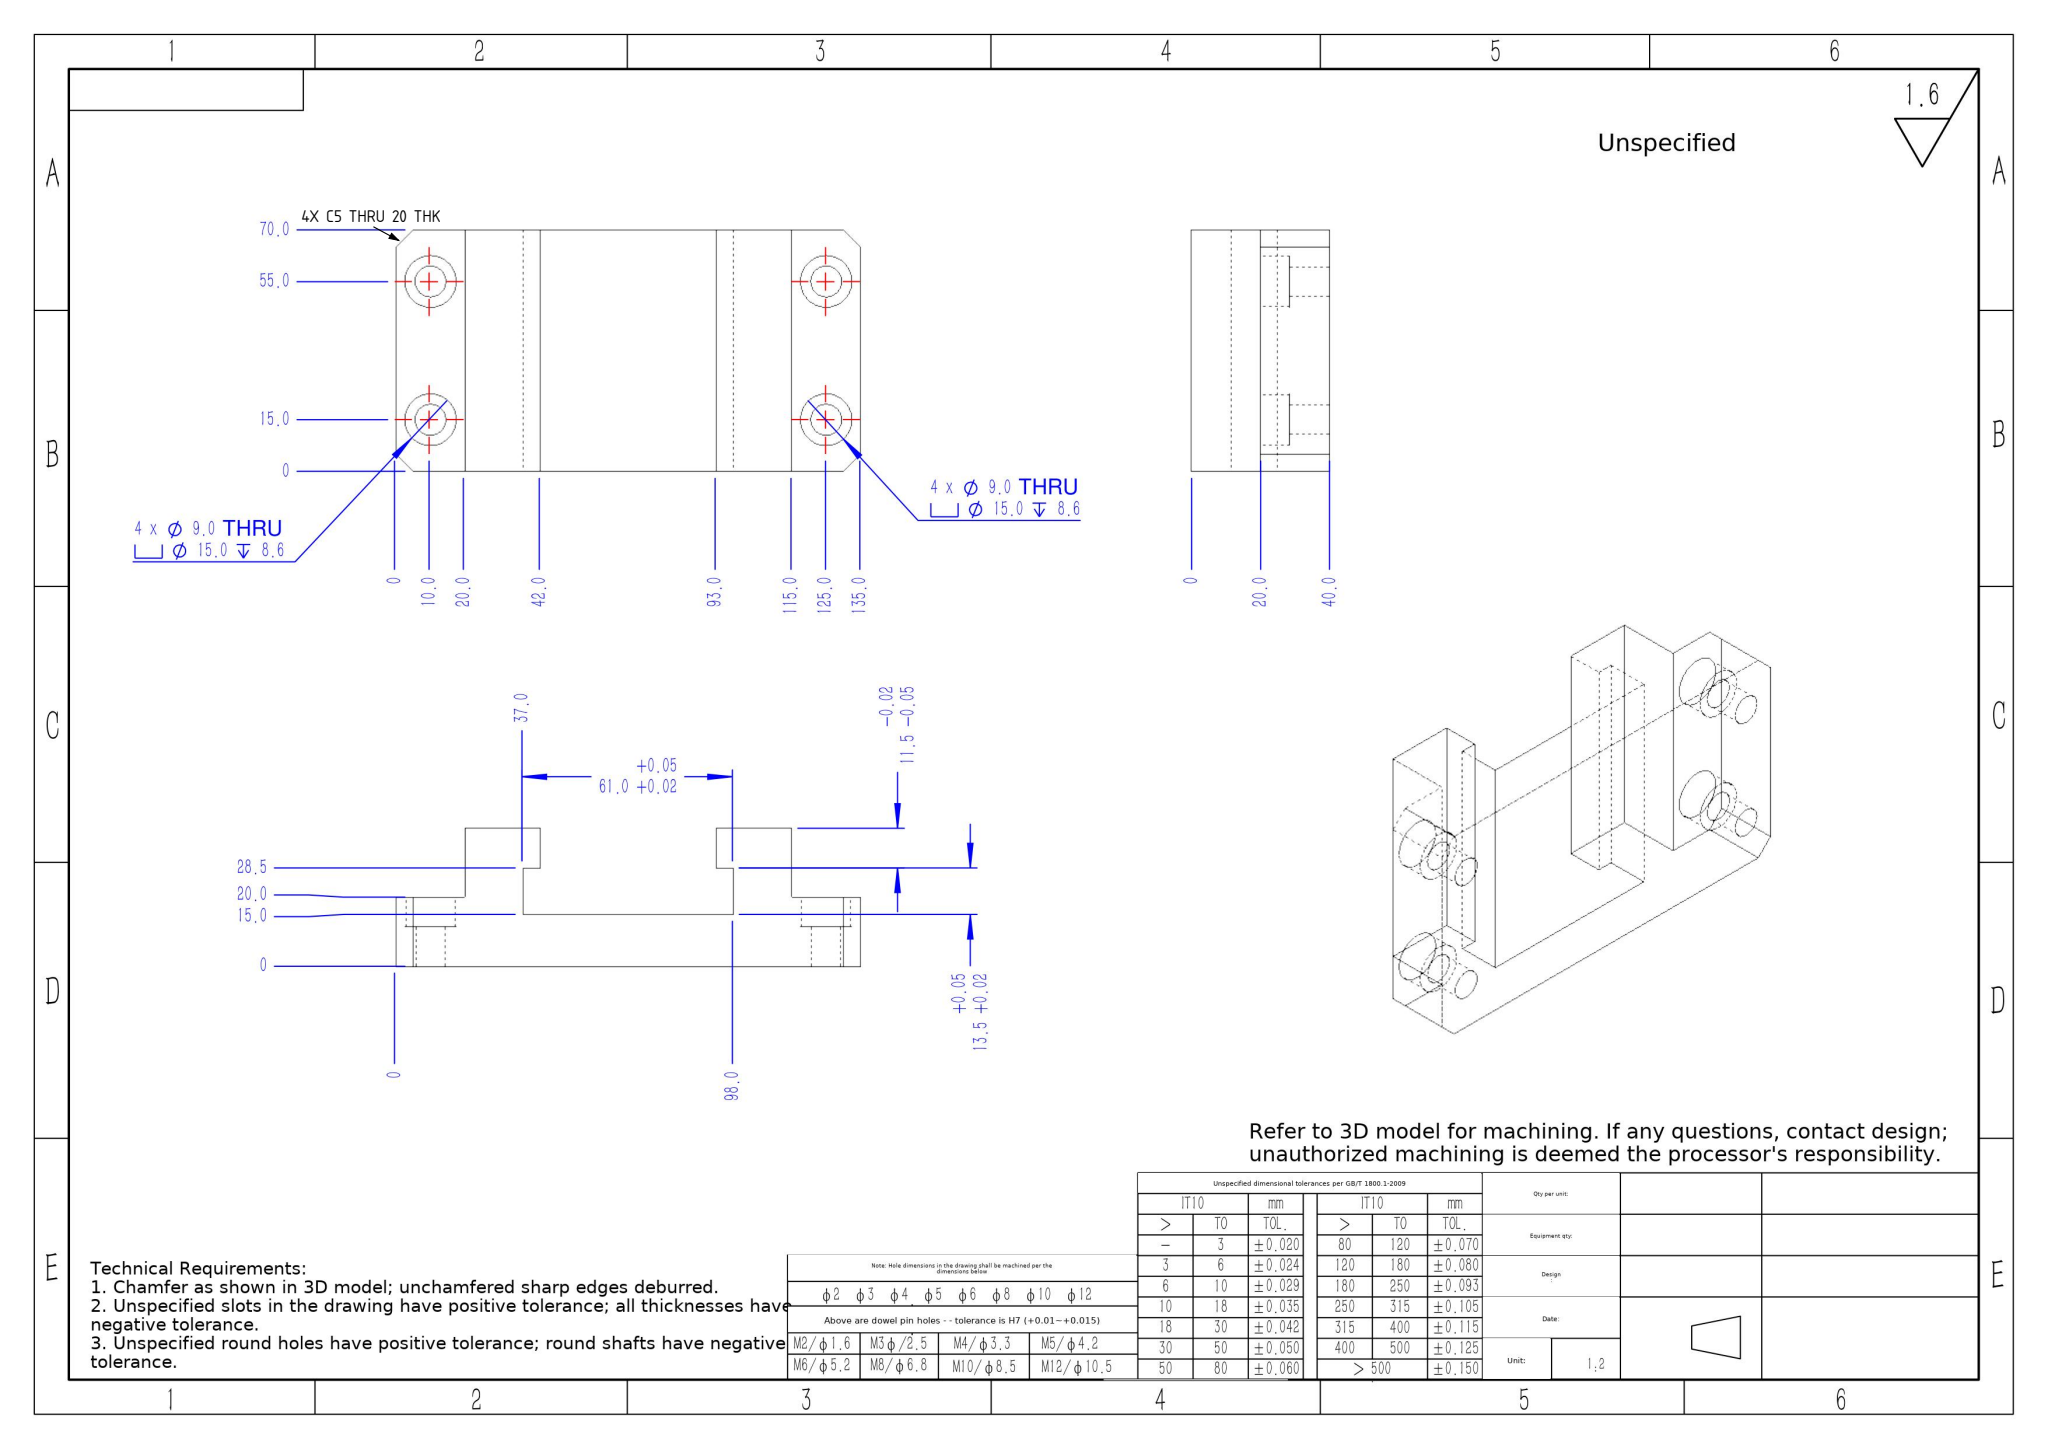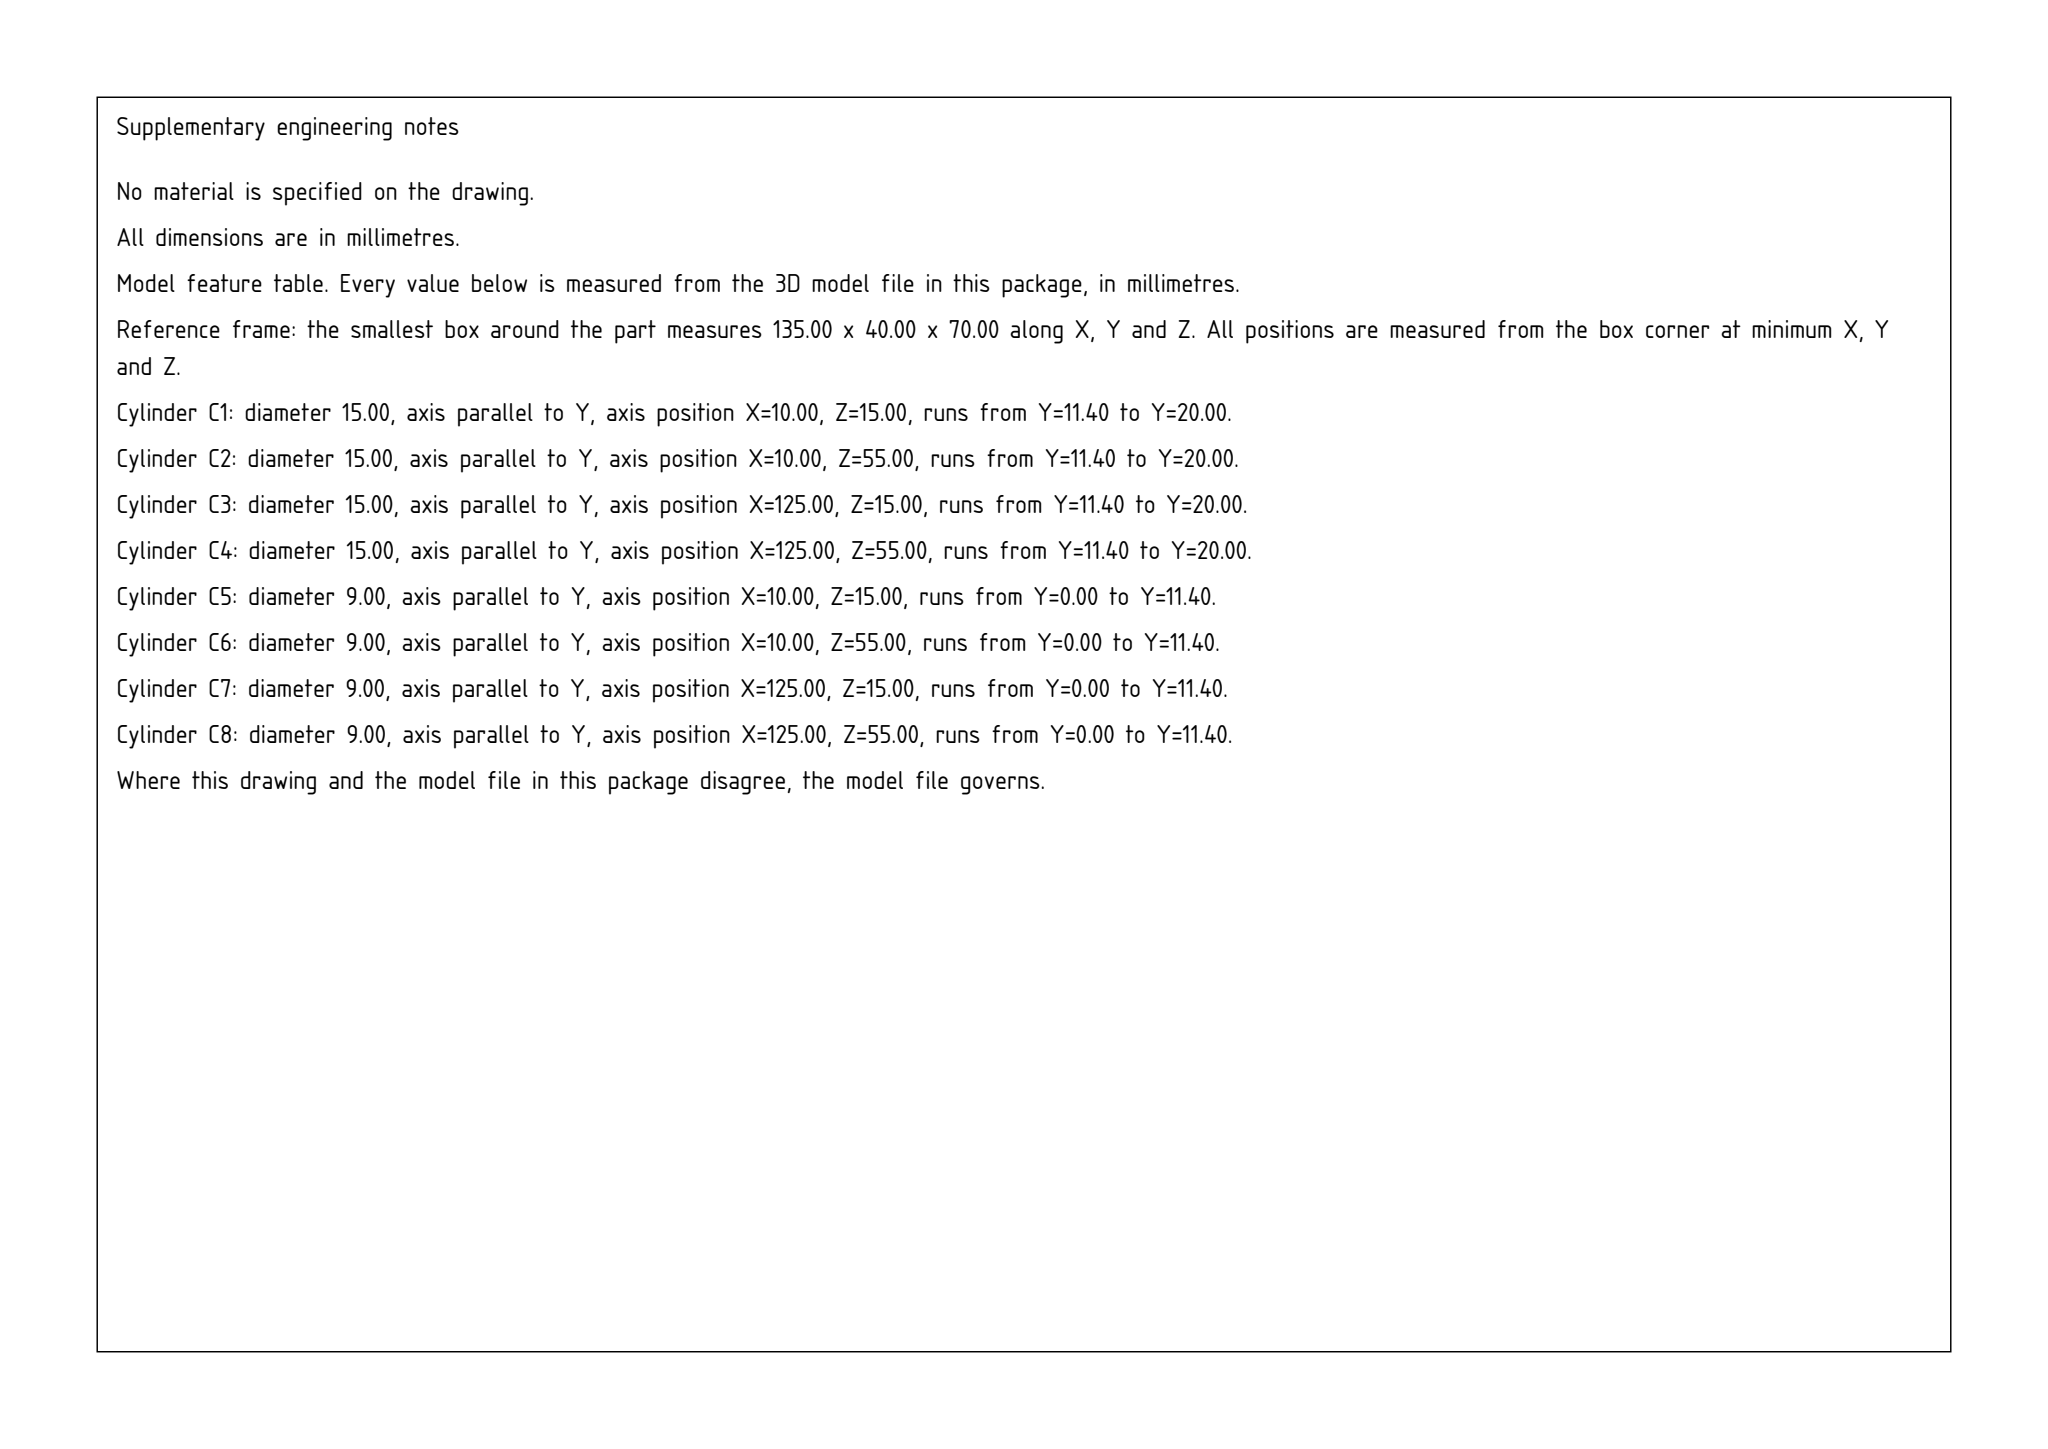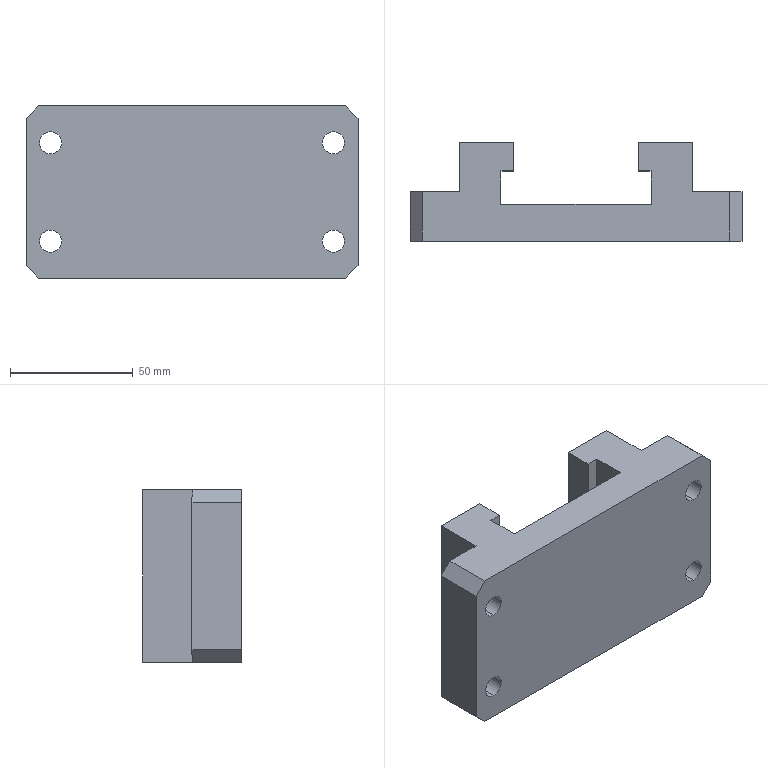Part | SolidWorks | mm | 1 solid | 42 faces | box 135 x 40 x 70 mm | volume 213320 mm3 | plane 26 | cylinder 16 | commonest cylinder face diameters 15 x8 9 x8
Drawing notes:
4X CHAMFER 5 x 45 deg on the four long corner edges of the lower plate (at X=0 and X=135 with Z=0 and Z=70), running full 20 mm thickness from Y=0 to Y=20. | from the solid: inclined_planes: angle_to_xyz_axes [45.0,90.0,45.0], bbox_from [0,0,0] / [0,0,65] / [130,0,0] / [130,0,65], size [5.0,20.0,5.0] (4 instances)
build123d program:
from build123d import *

# Parameters (mm, degrees)
SKETCH1_W                                       = 95
SKETCH1_H                                       = 70
BOSS_EXTRUDE1_DEPTH                             = 40
CUT_EXTRUDE1_DEPTH                              = 94.575
SKETCH3_W                                       = 70
SKETCH3_H                                       = 20
BOSS_EXTRUDE2_DEPTH                             = 20
M8_HEX_SOCKET_HEAD_CAP_SCREW_CBORE1_D           = 9
M8_HEX_SOCKET_HEAD_CAP_SCREW_CBORE1_CBORE_D     = 15
M8_HEX_SOCKET_HEAD_CAP_SCREW_CBORE1_CBORE_DEPTH = 8.6
MIRROR4_COPY_1_D                                = 9
MIRROR4_COPY_1_CBORE_D                          = 15
MIRROR4_COPY_1_CBORE_DEPTH                      = 8.6
CHAMFER1_SIZE                                   = 5


with BuildPart() as part:
    # Sketch1 → Boss-Extrude1 (new body)
    with BuildSketch(Plane(origin=(0, 0, 0), x_dir=(1, 0, 0), z_dir=(0, 1, 0))):
        Rectangle(SKETCH1_W, SKETCH1_H)
    extrude(amount=BOSS_EXTRUDE1_DEPTH)

    # Sketch2 → Cut-Extrude1 (cut, through all)
    with BuildSketch(Plane.XY.offset(35)):
        Polygon((-25.5, 40), (-25.5, 28.5), (-30.5, 28.5), (-30.5, 15), (30.5, 15), (30.5, 28.5), (25.5, 28.5), (25.5, 40), align=None)
    extrude(amount=-CUT_EXTRUDE1_DEPTH, mode=Mode.SUBTRACT)

    # Sketch3 → Boss-Extrude2 (add)
    with BuildSketch(Plane(origin=(47.5, 0, 0), x_dir=(0, 0, -1), z_dir=(1, 0, 0))):
        with Locations((0, 10)):
            Rectangle(SKETCH3_W, SKETCH3_H)
    boss_extrude2 = extrude(amount=BOSS_EXTRUDE2_DEPTH)

    # Mirror1: Boss-Extrude2 across plane
    add(boss_extrude2.mirror(Plane(origin=(0, 0, 0), x_dir=(0, 0, 1), z_dir=(1, 0, 0))))

    # M8 Hex Socket Head Cap Screw CBORE1 (through all)
    with Locations(Plane(origin=(0, 20, 0), x_dir=(1, 0, 0), z_dir=(0, 1, 0))):
        with Locations((-57.5, -20)):
            m8_hex_socket_head_cap_screw_cbore1 = CounterBoreHole(M8_HEX_SOCKET_HEAD_CAP_SCREW_CBORE1_D / 2, M8_HEX_SOCKET_HEAD_CAP_SCREW_CBORE1_CBORE_D / 2, M8_HEX_SOCKET_HEAD_CAP_SCREW_CBORE1_CBORE_DEPTH)

    # Mirror3: M8 Hex Socket Head Cap Screw CBORE1 across plane
    add(m8_hex_socket_head_cap_screw_cbore1.mirror(Plane.XY), mode=Mode.SUBTRACT)

    # Mirror4: M8 Hex Socket Head Cap Screw CBORE1 across plane
    add(m8_hex_socket_head_cap_screw_cbore1.mirror(Plane(origin=(0, 0, 0), x_dir=(0, 0, 1), z_dir=(1, 0, 0))), mode=Mode.SUBTRACT)

    # Mirror4 copy 1 (through all)
    with Locations(Plane(origin=(0, 20, 0), x_dir=(-1, 0, 0), z_dir=(0, 1, 0))):
        with Locations((-57.5, -20)):
            CounterBoreHole(MIRROR4_COPY_1_D / 2, MIRROR4_COPY_1_CBORE_D / 2, MIRROR4_COPY_1_CBORE_DEPTH)

    # Chamfer1
    chamfer1_edges = [part.edges().sort_by_distance(p)[0] for p in [
        (67.5, 10, 35),
        (67.5, 10, -35),
        (-67.5, 10, 35),
        (-67.5, 10, -35),
    ]]
    chamfer(chamfer1_edges, length=CHAMFER1_SIZE)


solid = part.part